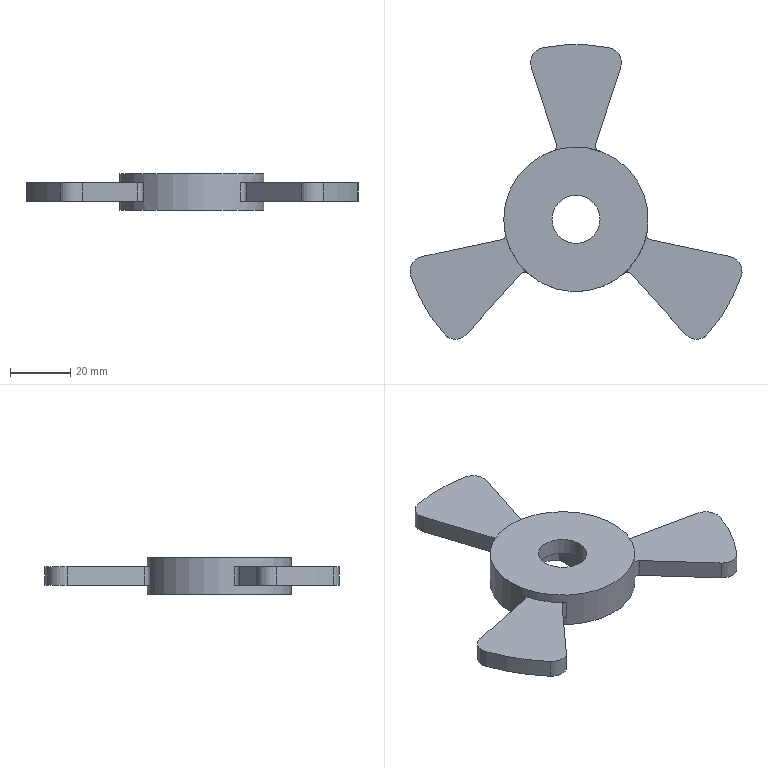Component | NX | IMPELLER | 1 solid | 36 faces | volume 31571 mm3 | cylinder 19 | plane 17 | commonest cylinder face diameters 10 x6 3 x6 116 x3 25 x2 48 x1 16 x1